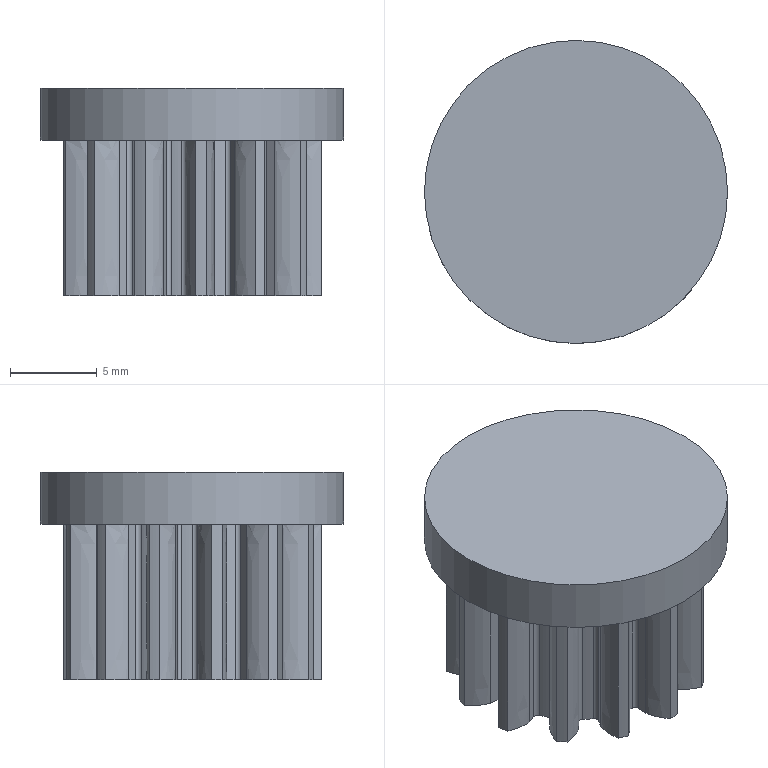Component | NX | BASE-GEAR-YENI | 1 solid | 108 faces | volume 1871 mm3 | cylinder 53 | plane 29 | other 26 | commonest cylinder face diameters 0.5 x26 15 x13 10.5 x13 17.5 x1